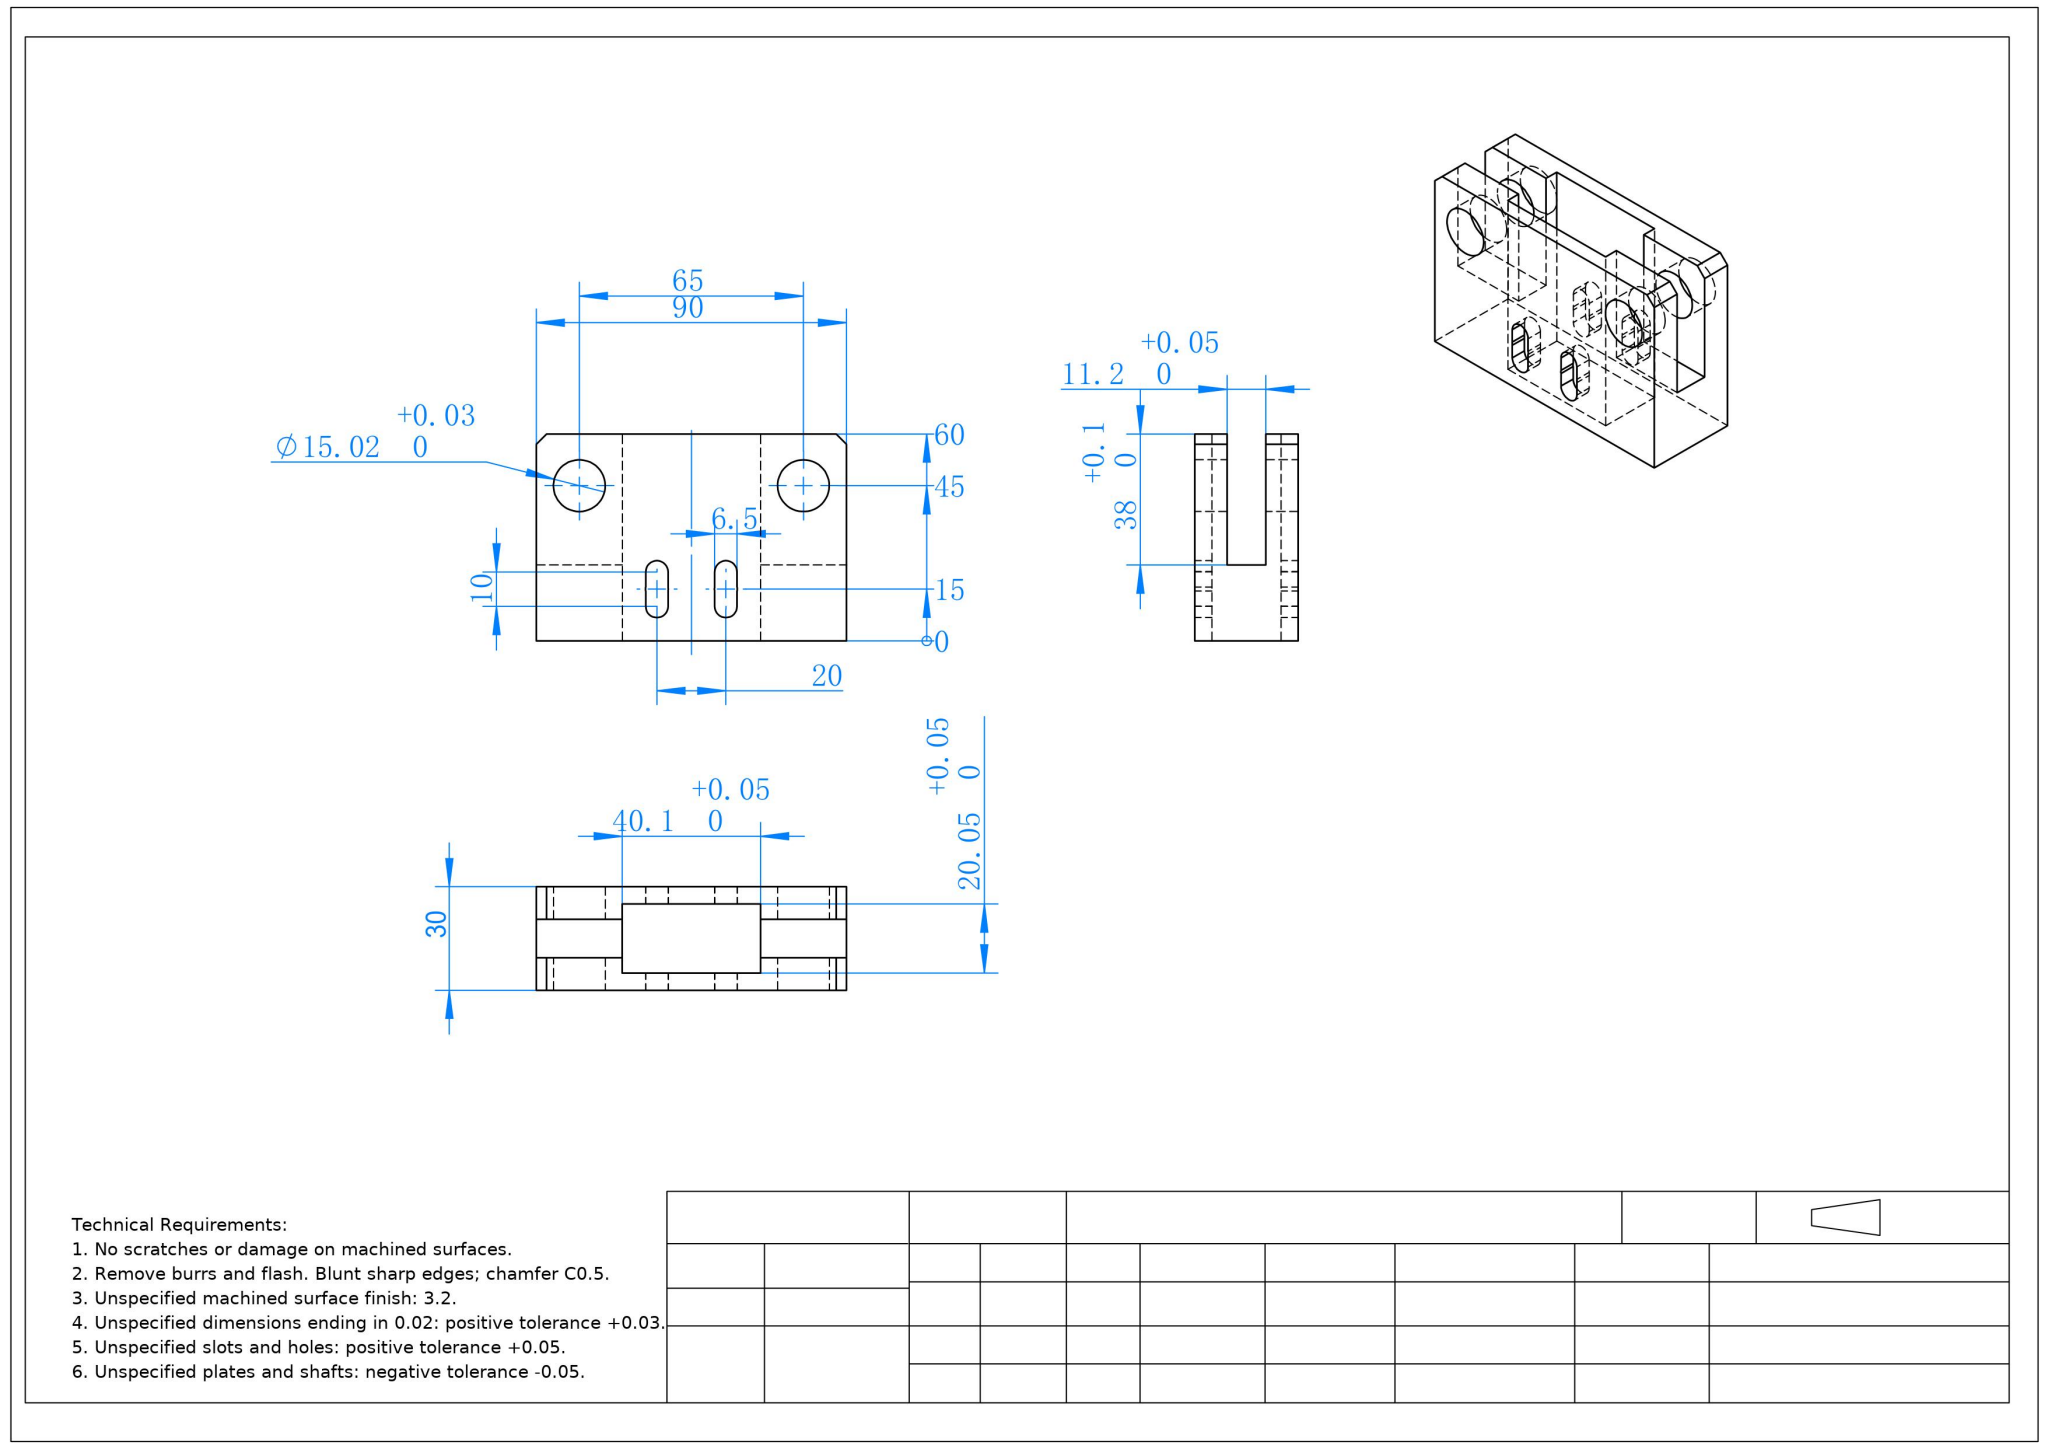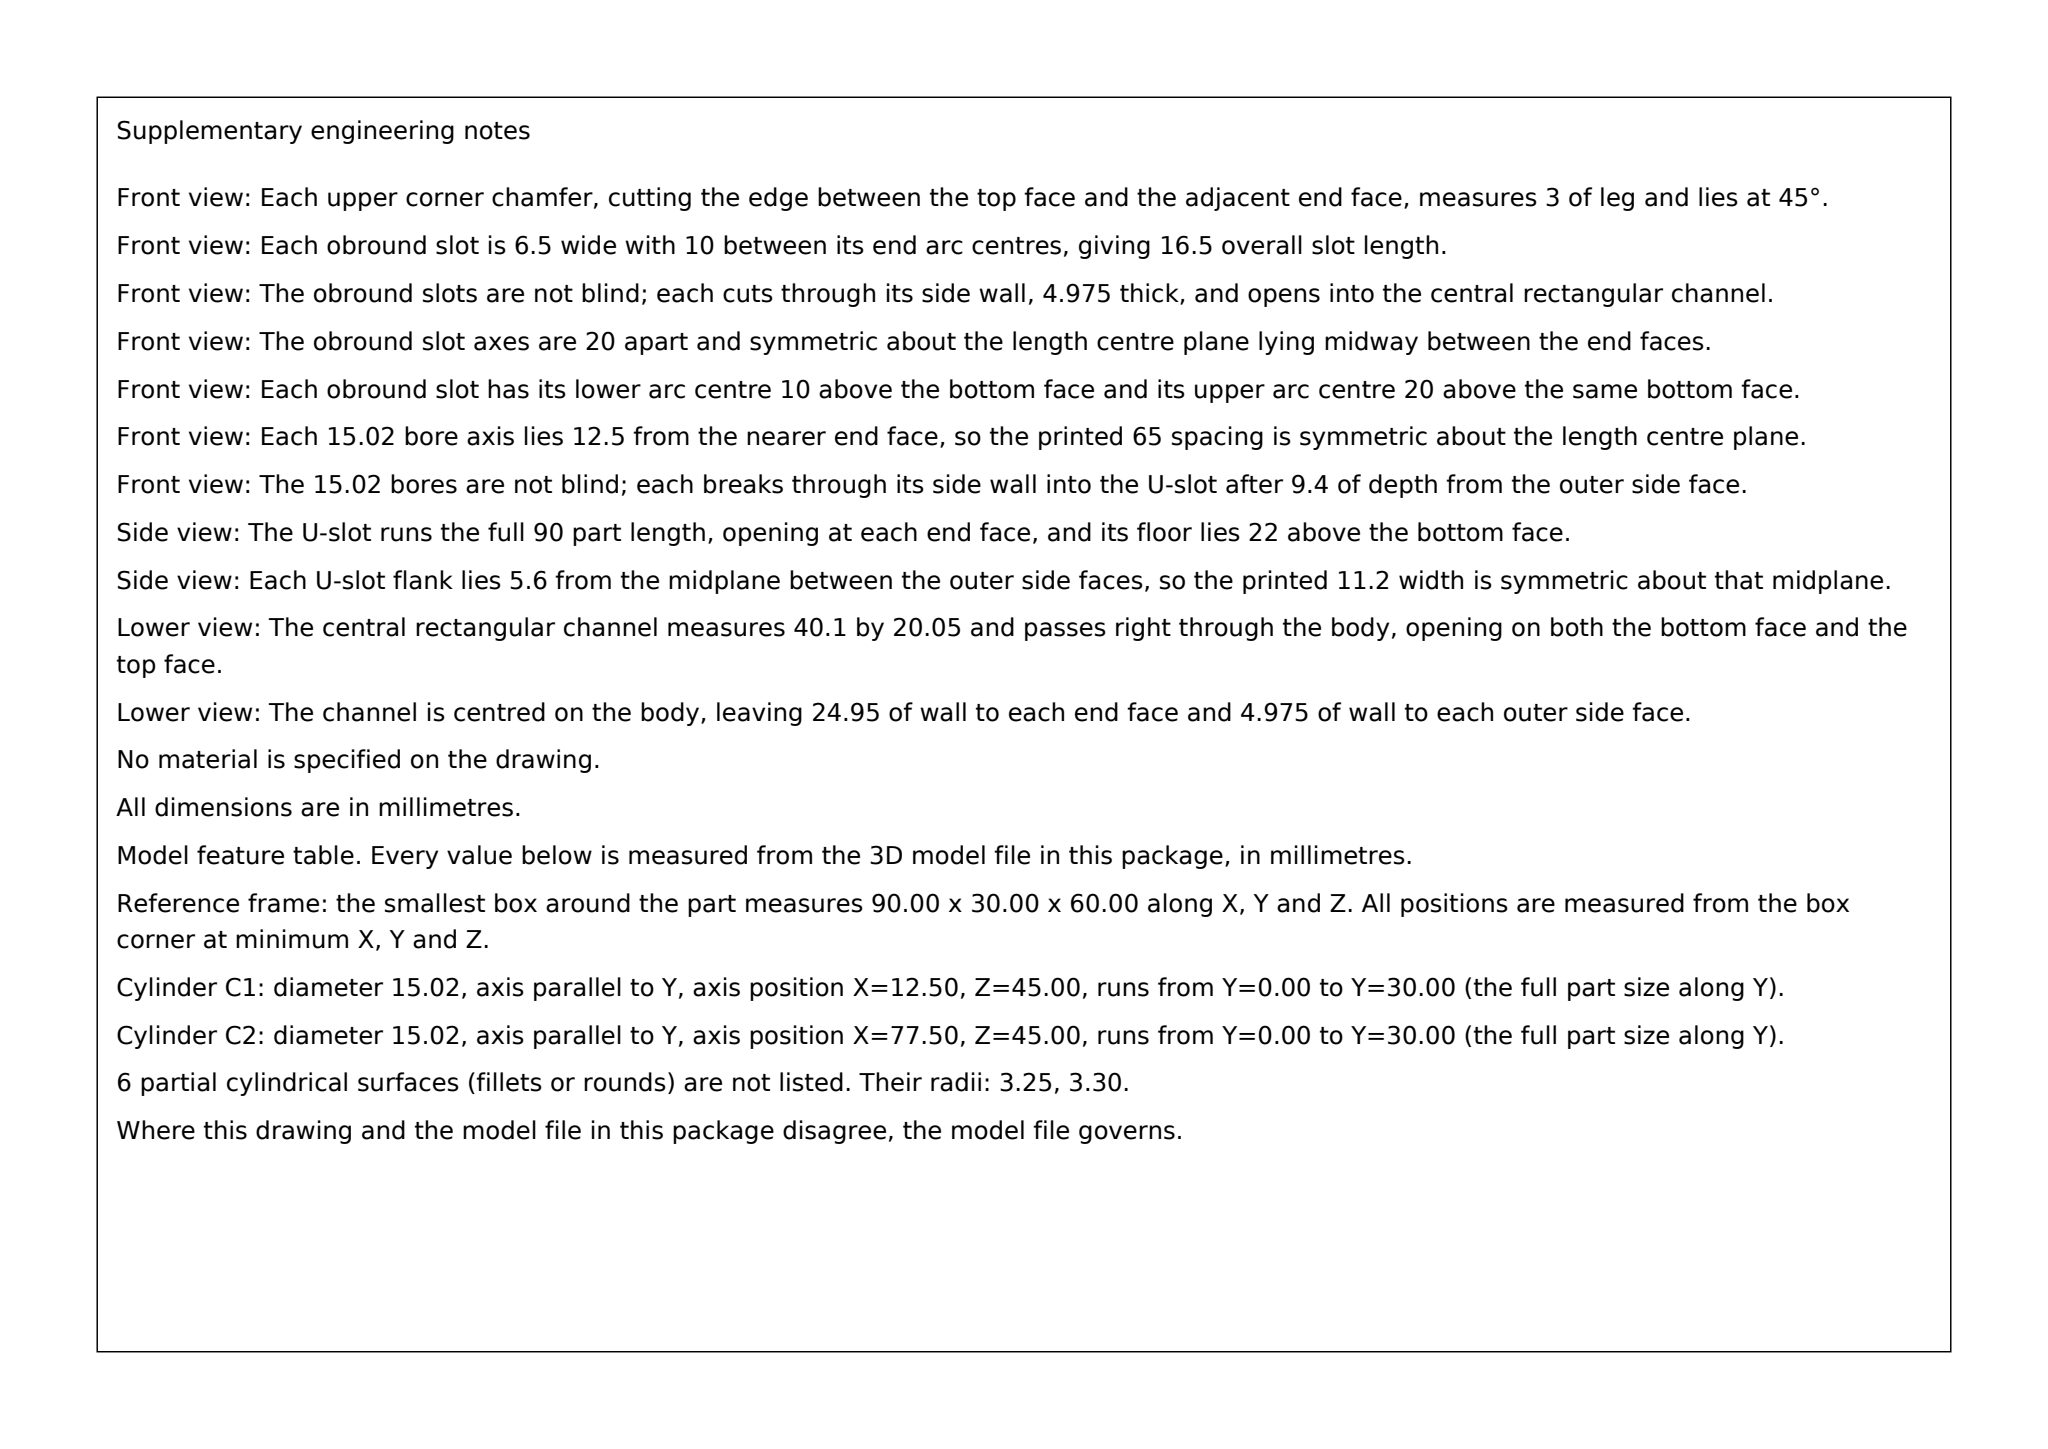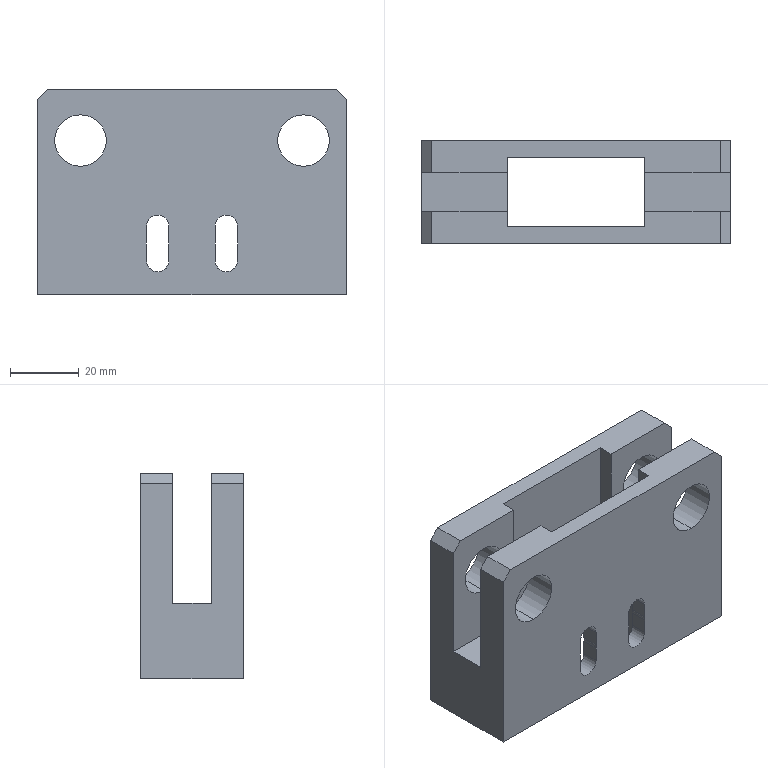Part | SolidWorks | mm | 1 solid | 65 faces | box 90 x 30 x 60 mm | volume 83735 mm3 | plane 37 | cylinder 28 | commonest cylinder face diameters 6.5 x12 15.02 x8 6.6 x8
build123d program:
from build123d import *

# Parameters (mm, degrees)
SKETCH1_W            = 90
SKETCH1_H            = 30
BOSS_EXTRUDE1_DEPTH  = 60
SKETCH2_W            = 90
SKETCH2_H            = 11.2
CUT_EXTRUDE1_DEPTH   = 38
SKETCH3_R            = 7.51
CUT_EXTRUDE2_DEPTH   = 81.777
CHAMFER1_SIZE        = 3
SKETCH4_W            = 40.1
SKETCH4_H            = 20.05
CUT_EXTRUDE3_DEPTH   = 77.485
M7_CLEARANCE_HOLE1_D = 6.6
CUT_EXTRUDE4_DEPTH   = 81.777


with BuildPart() as part:
    # Sketch1 → Boss-Extrude1 (new body)
    with BuildSketch(Plane.XY):
        Rectangle(SKETCH1_W, SKETCH1_H)
    extrude(amount=BOSS_EXTRUDE1_DEPTH)

    # Sketch2 → Cut-Extrude1 (cut)
    with BuildSketch(Plane.XY.offset(60)):
        Rectangle(SKETCH2_W, SKETCH2_H)
    extrude(amount=-CUT_EXTRUDE1_DEPTH, mode=Mode.SUBTRACT)

    # Sketch3 → Cut-Extrude2 (cut, through all)
    with BuildSketch(Plane.XZ.offset(15)):
        with Locations(Location((-32.5, 45, 0), (0, 0, 270))):
            Circle(SKETCH3_R)
        with Locations((32.5, 45)):
            Circle(SKETCH3_R)
    extrude(amount=-CUT_EXTRUDE2_DEPTH, mode=Mode.SUBTRACT)

    # Chamfer1
    chamfer1_edges = [part.edges().sort_by_distance(p)[0] for p in [
        (45, -10.3, 60),
        (-45, -10.3, 60),
        (45, 10.3, 60),
        (-45, 10.3, 60),
    ]]
    chamfer(chamfer1_edges, length=CHAMFER1_SIZE)

    # Sketch4 → Cut-Extrude3 (cut, through all)
    with BuildSketch(Plane.XY.offset(60)):
        Rectangle(SKETCH4_W, SKETCH4_H)
    extrude(amount=-CUT_EXTRUDE3_DEPTH, mode=Mode.SUBTRACT)

    # M7 Clearance Hole1 (through all)
    with Locations(Plane(origin=(0, -15, 0), x_dir=(-1, 0, 0), z_dir=(0, -1, 0))):
        with Locations((10, -15), (-10, -15)):
            Hole(M7_CLEARANCE_HOLE1_D / 2)

    # Sketch8 → Cut-Extrude4 (cut, through all)
    with BuildSketch(Plane(origin=(0, 15, 0), x_dir=(1, 0, 0), z_dir=(0, 1, 0))):
        with BuildLine():
            Line((-13.25, -20), (-13.25, -10))
            ThreePointArc((-13.25, -10), (-10, -6.75), (-6.75, -10))
            Line((-6.75, -10), (-6.75, -20))
            ThreePointArc((-6.75, -20), (-10, -23.25), (-13.25, -20))
        make_face()
        with BuildLine():
            Line((6.75, -20), (6.75, -10))
            ThreePointArc((6.75, -10), (10, -6.75), (13.25, -10))
            Line((13.25, -10), (13.25, -20))
            ThreePointArc((13.25, -20), (10, -23.25), (6.75, -20))
        make_face()
    extrude(amount=-CUT_EXTRUDE4_DEPTH, mode=Mode.SUBTRACT)


solid = part.part